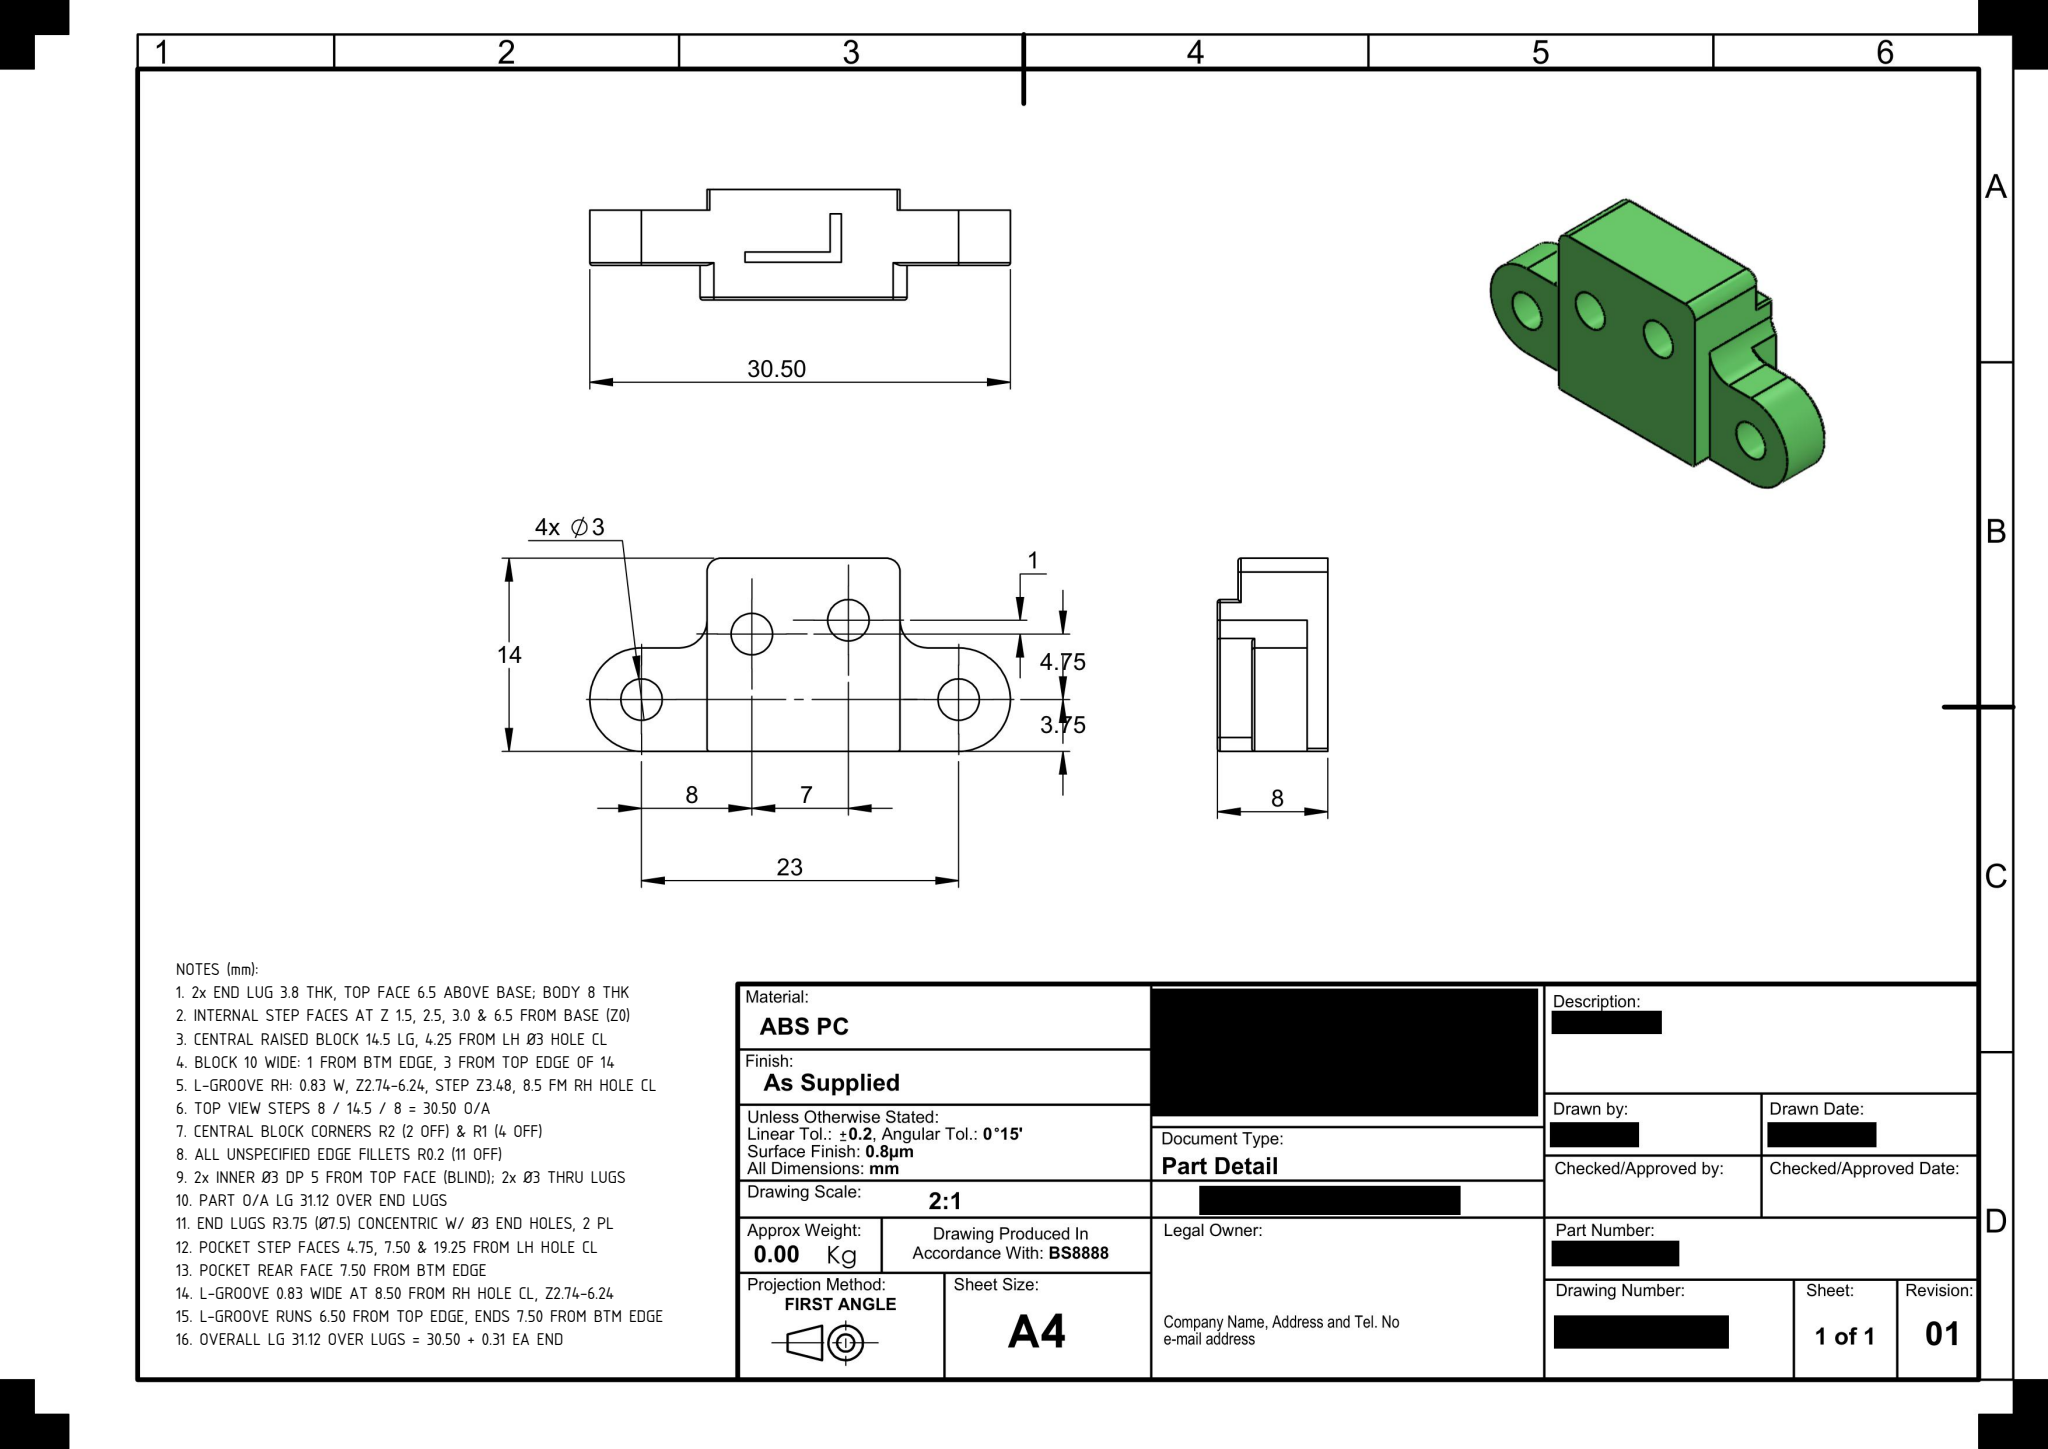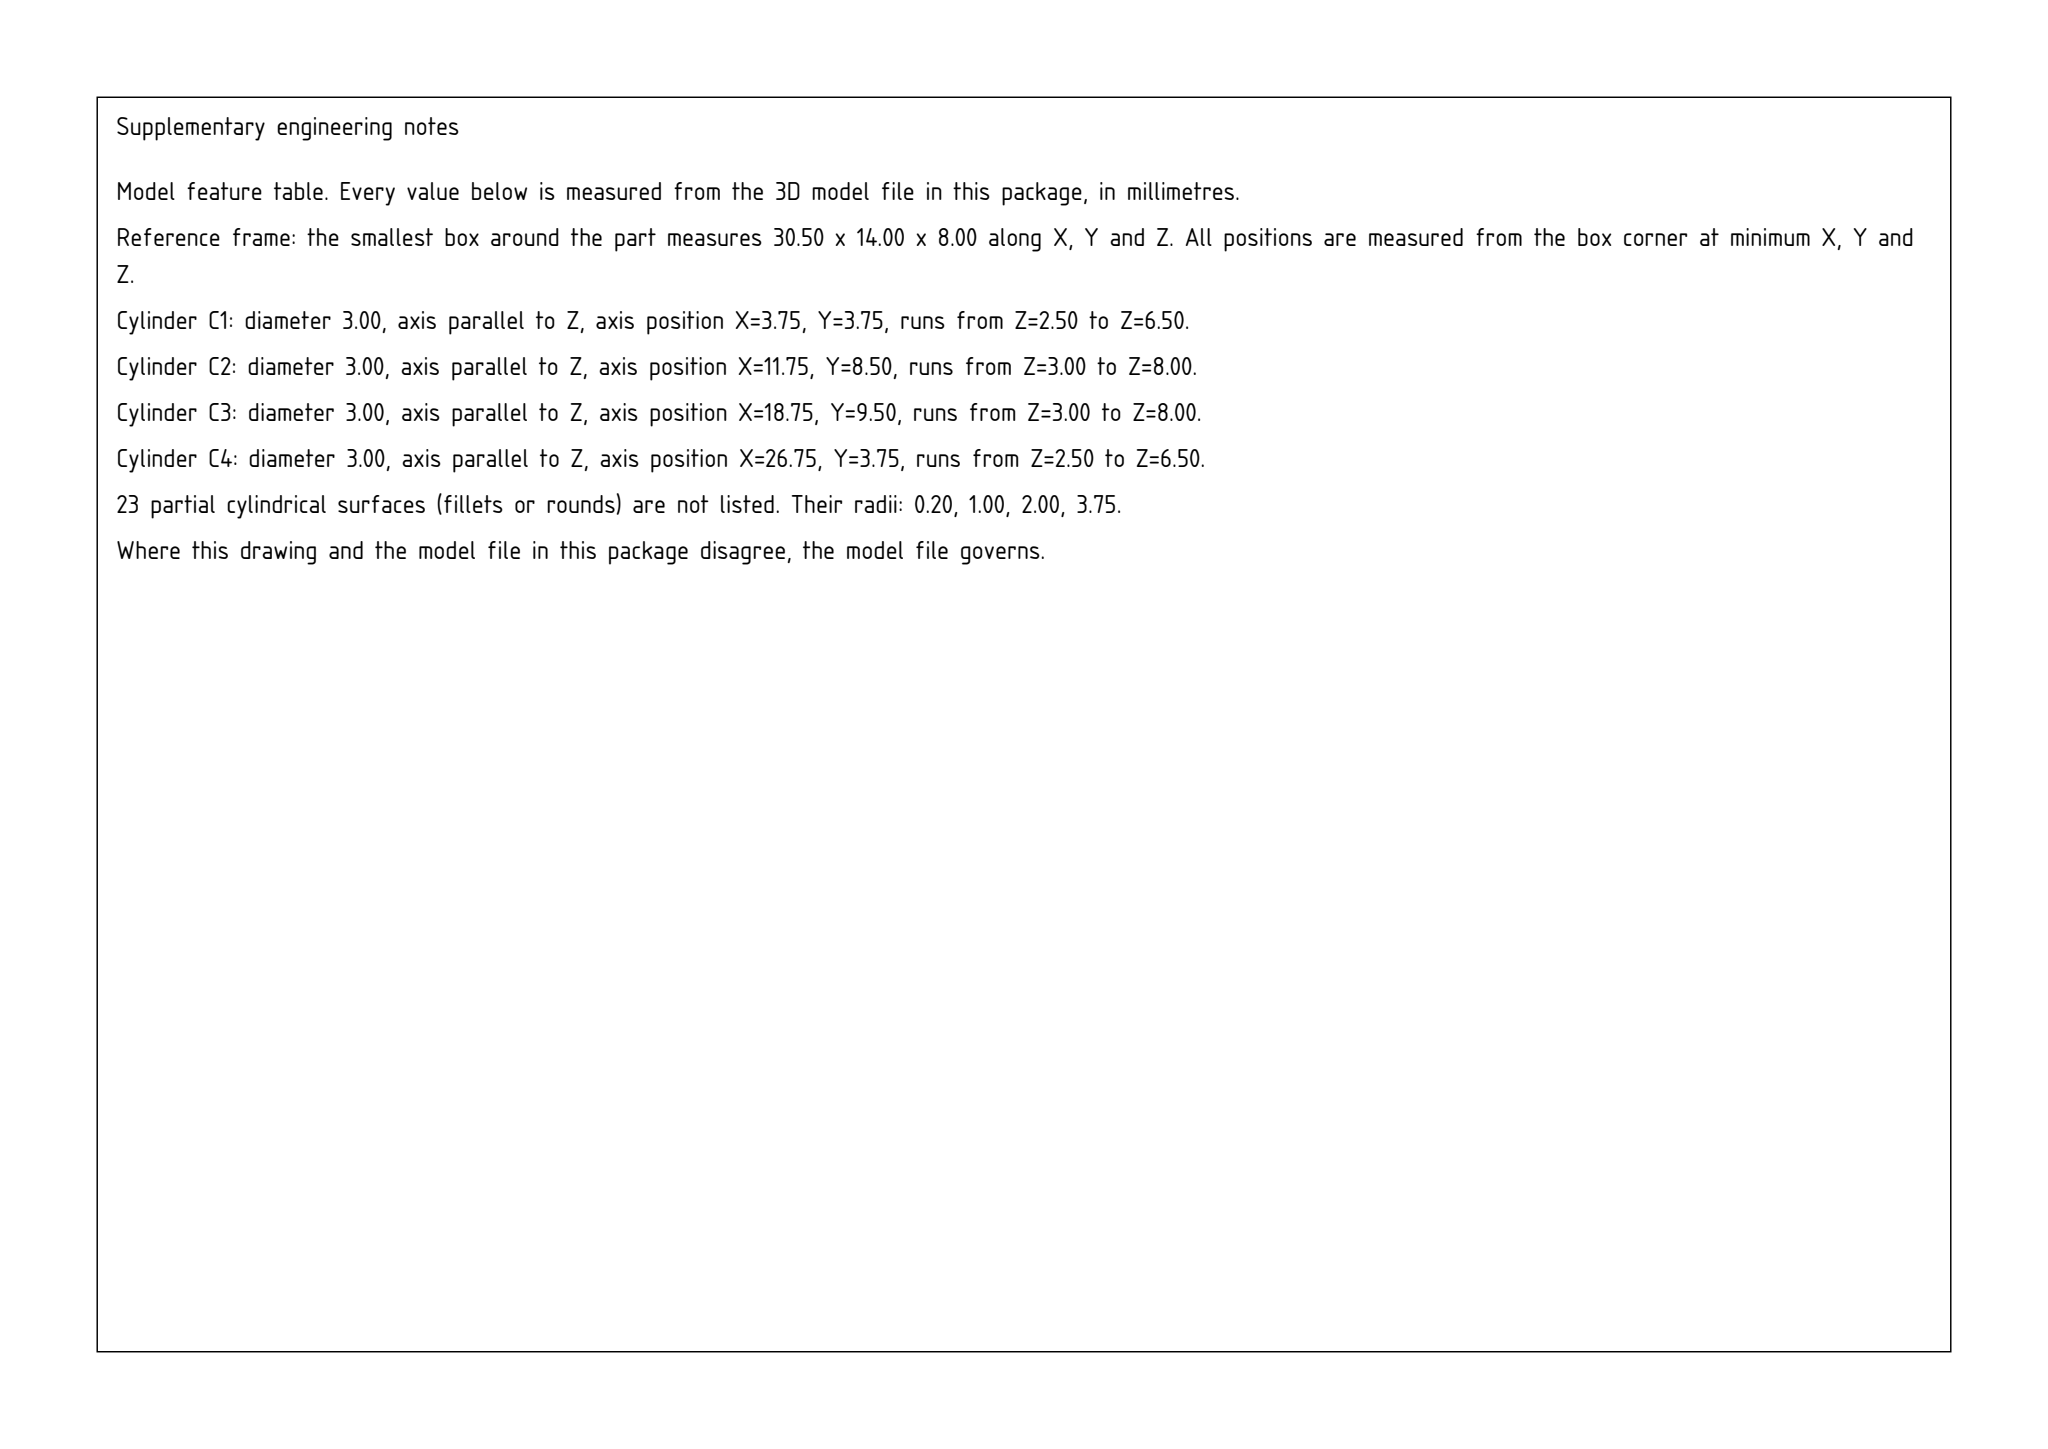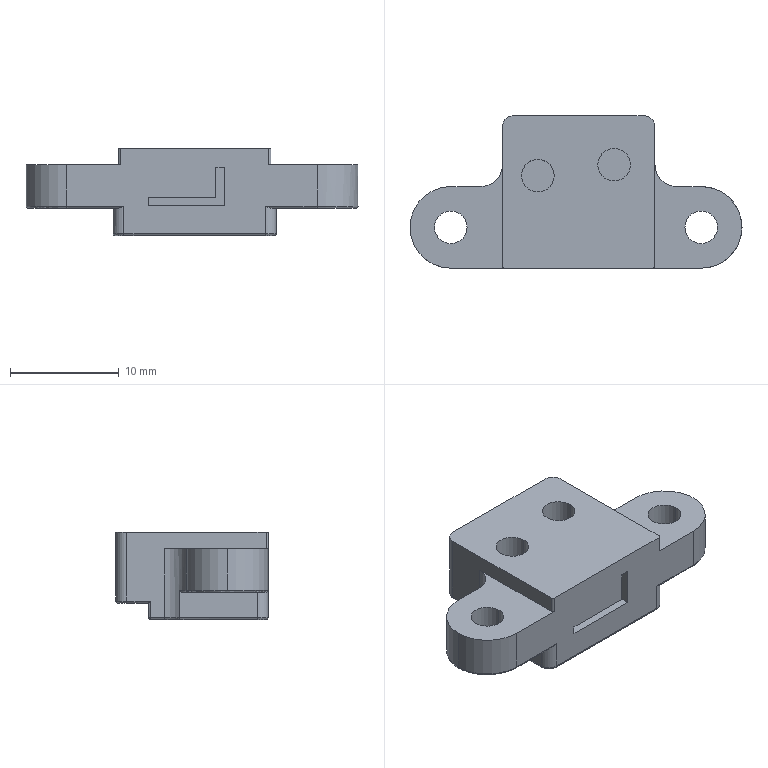Part | SolidWorks | mm | 1 solid | 72 faces | box 30.5 x 14 x 8 mm | volume 1840 mm3 | cylinder 34 | plane 25 | torus 11 | sphere 2 | commonest cylinder face diameters 0.4 x17 3 x8 2 x4 7.5 x3 4 x2
Drawing notes:
2x END LUG 3.8 THK, TOP FACE 6.5 ABOVE BASE; BODY 8 THK | from the solid: Ø7.5 z-cyl len 3.8 at (4.06,4.06) & (27.06,4.06); z planes 6.5 & 8.0; bbox z=8.0
INTERNAL STEP FACES AT Z 1.5, 2.5, 3.0 & 6.5 FROM BASE (Z0) | from the solid: axis_planes z: 0, 1.5, 2.5(x2), 3.0(x2), 6.5(x2), 8.0
CENTRAL RAISED BLOCK 14.5 LG, 4.25 FROM LH Ø3 HOLE CL | from the solid: x planes 8.31 & 22.81 (14.5); LH lug hole CL x=4.06, 8.31-4.06=4.25
BLOCK 10 WIDE: 1 FROM BTM EDGE, 3 FROM TOP EDGE OF 14 | from the solid: y planes 1.31 & 11.31 (10 wide) within y 0.31-14.31 (14 O/A)
L-GROOVE RH: 0.83 W, Z2.74-6.24, STEP Z3.48, 8.5 FM RH HOLE CL | from the solid: x planes 17.73/18.56 (0.83); z planes 2.74/3.48/6.24; RH hole CL x=27.06, 27.06-18.56=8.5
TOP VIEW STEPS 8 / 14.5 / 8 = 30.50 O/A | from the solid: lug ends x=0.31 & 30.81; block faces x=8.31 & 22.81
CENTRAL BLOCK CORNERS R2 (2 OFF) & R1 (4 OFF) | from the solid: Ø4 z-cyls at (6.81,9.81),(24.81,9.81)=R2; Ø2 z-cyls at (9.31,1.31),(22.31,1.31),(9.81,13.31),(21.81,13.31)=R1
ALL UNSPECIFIED EDGE FILLETS R0.2 (11 OFF) | from the solid: fillet_radii [[0.2,11]]
2x INNER Ø3 DP 5 FROM TOP FACE (BLIND); 2x Ø3 THRU LUGS | from the solid: Ø3 z-cyls len 5.0 at (12.06,8.81),(19.06,9.81), bottoms at z=3.0; Ø3 len 4.0 at lugs
PART O/A LG 31.12 OVER END LUGS | from the solid: bbox_xyz x = 31.118
END LUGS R3.75 (Ø7.5) CONCENTRIC W/ Ø3 END HOLES, 2 PL | from the solid: cylinders Ø7.5 z-axis at (4.06,4.06) & (27.06,4.06), same centres as Ø3 end holes; profile edges at x0.31/30.81, y0.31
POCKET STEP FACES 4.75, 7.50 & 19.25 FROM LH HOLE CL | from the solid: axis_planes x = 8.81, 11.56, 23.31 minus LH hole CL x=4.06
POCKET REAR FACE 7.50 FROM BTM EDGE | from the solid: axis_plane y = 7.81 minus bottom profile edge y = 0.31
L-GROOVE 0.83 WIDE AT 8.50 FROM RH HOLE CL, Z2.74-6.24 | from the solid: axis_planes x 17.73 & 18.56 (0.83 apart; 27.06-18.56=8.50); z planes 2.74, 3.48, 6.24
L-GROOVE RUNS 6.50 FROM TOP EDGE, ENDS 7.50 FROM BTM EDGE | from the solid: y planes 14.31 (top edge) to 7.81; 14.31-7.81=6.50, 7.81-0.31=7.50
OVERALL LG 31.12 OVER LUGS = 30.50 + 0.31 EA END | from the solid: bbox_x 31.118 vs lug-to-lug 30.50 (x 0.31 to 30.81); (31.118-30.50)/2=0.309